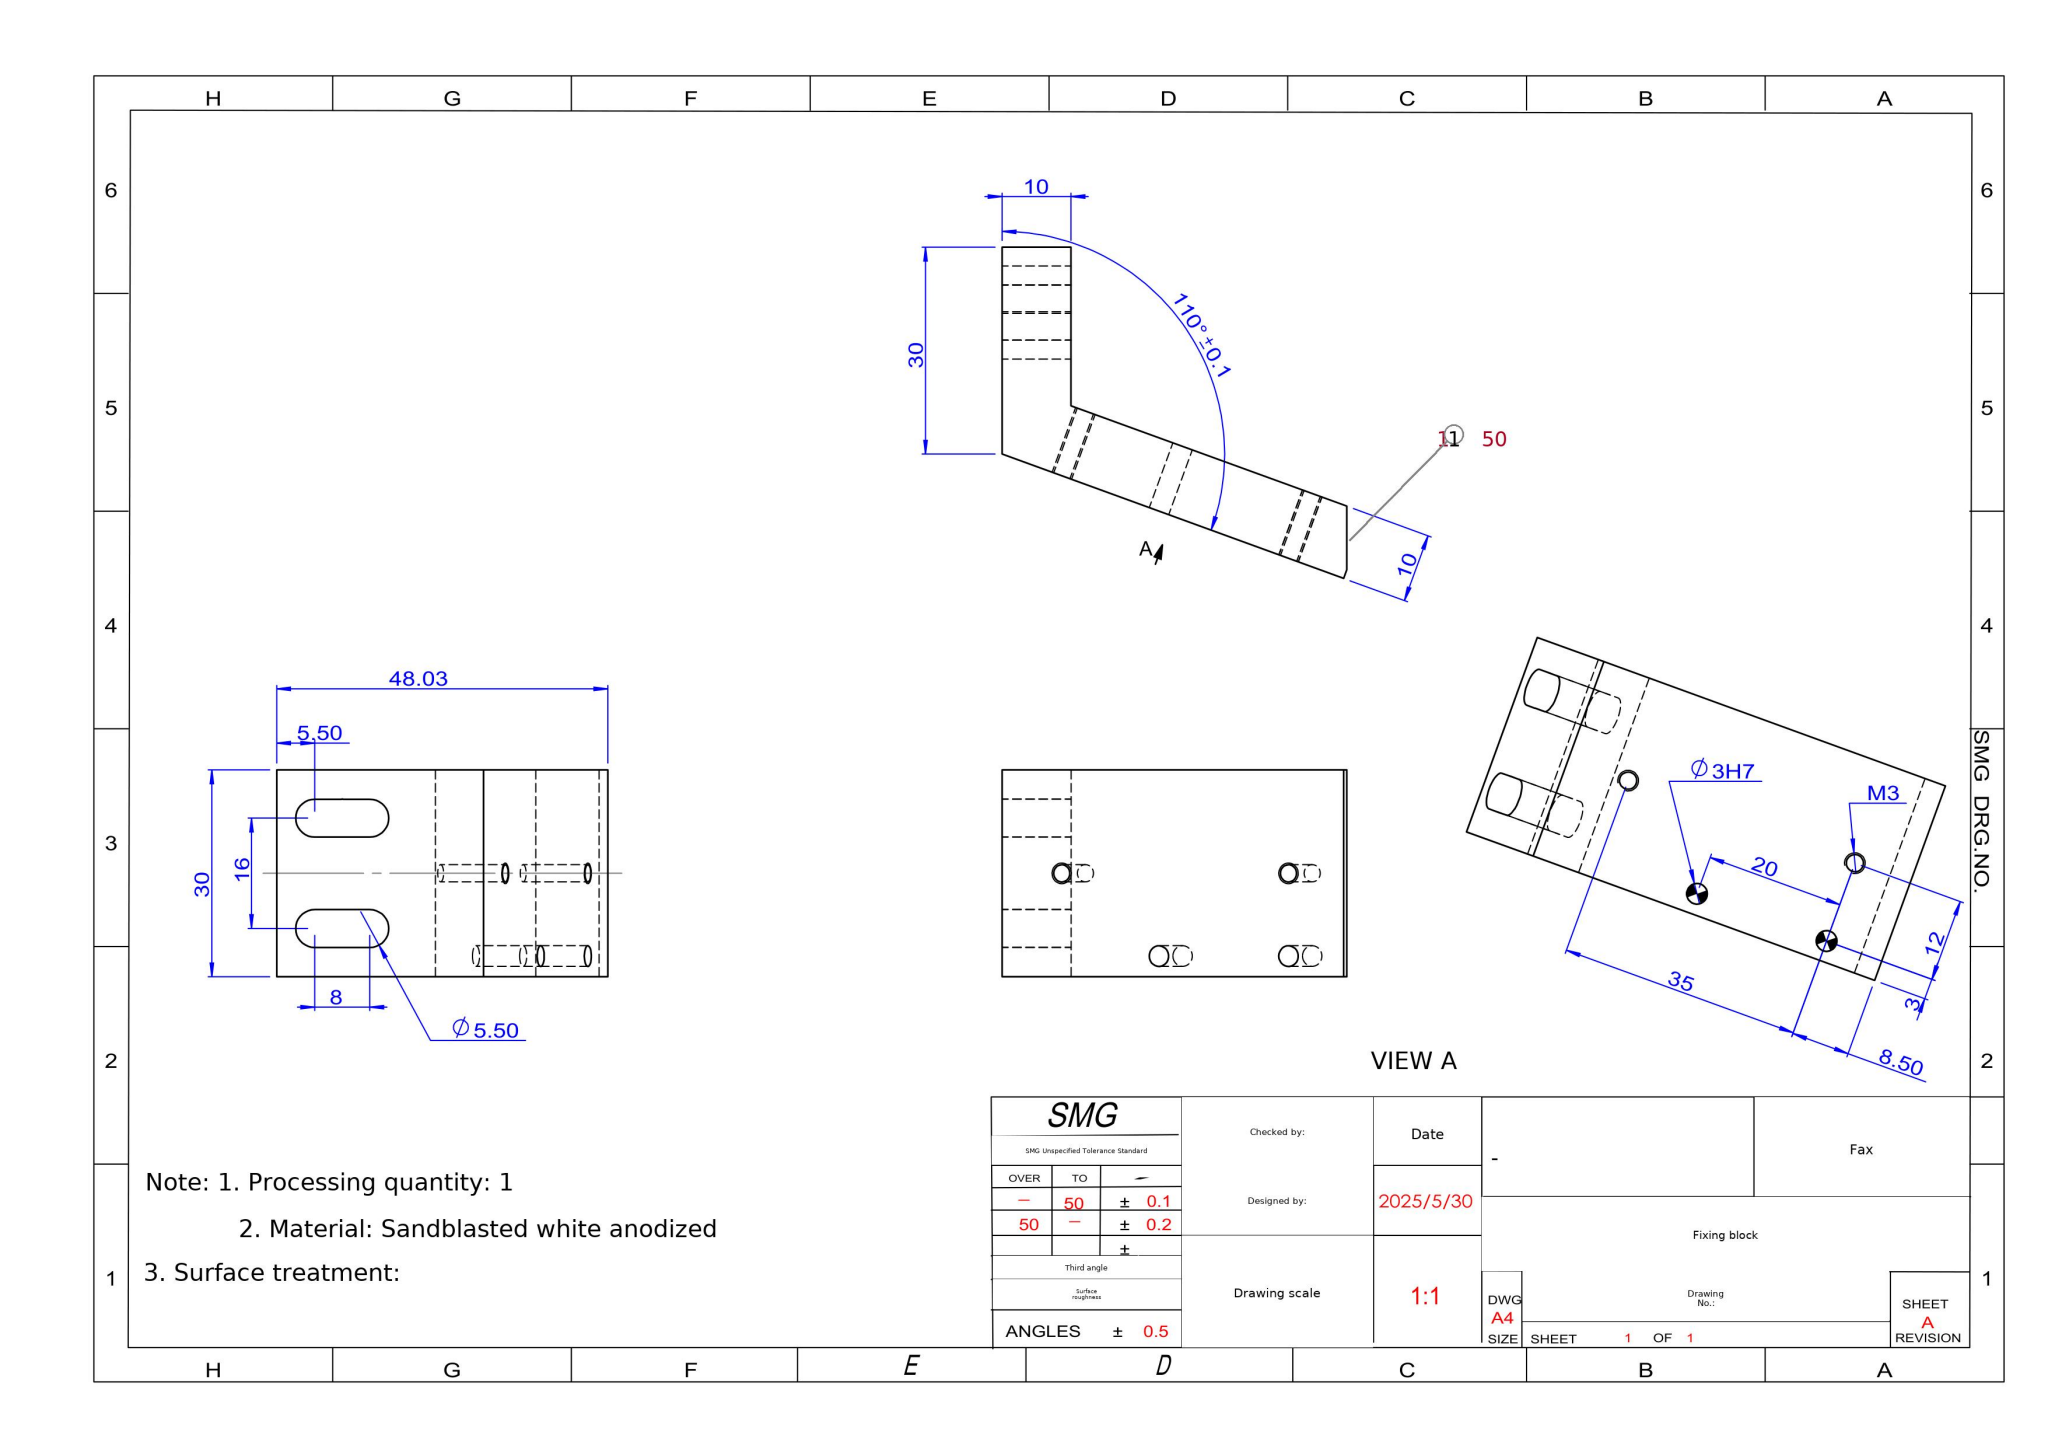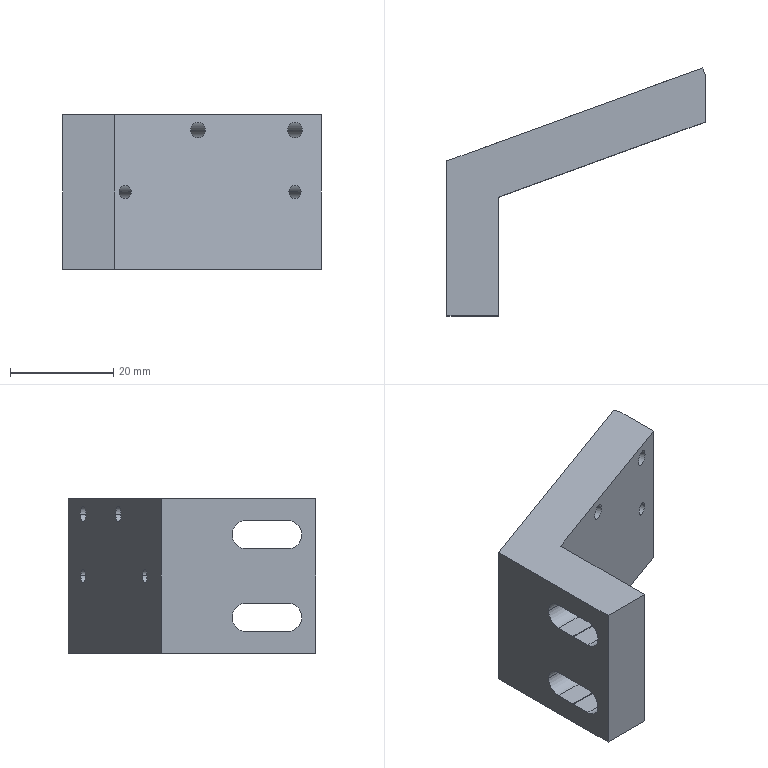Part | SolidWorks | mm | material Sandblasted white anodized | 1 solid | 35 faces | box 50 x 48.03 x 30 mm | volume 20713 mm3 | cylinder 18 | plane 17 | commonest cylinder face diameters 5.495 x6 2.5 x4 3 x4 5.5 x4